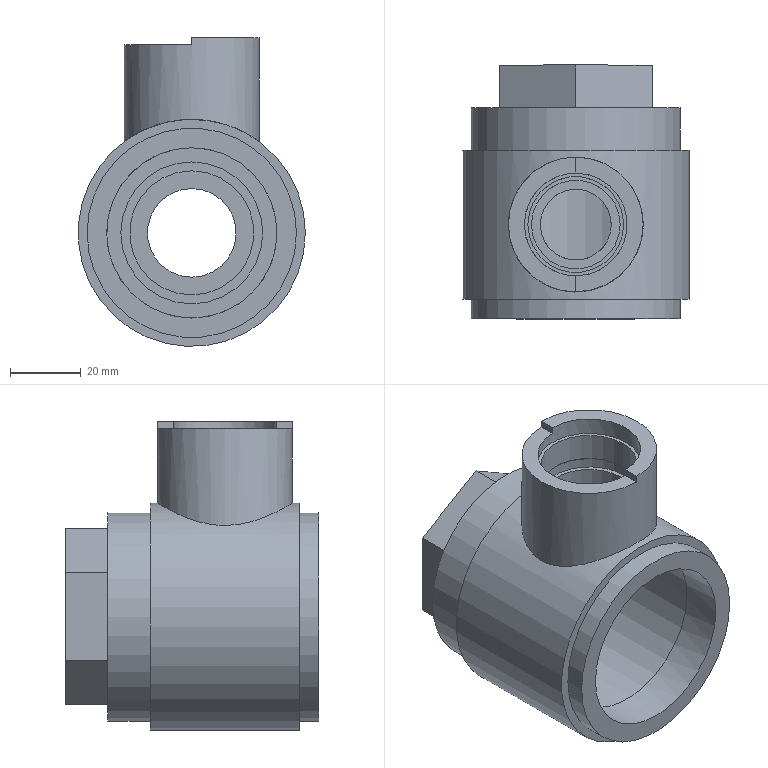Component | NX | VALVEBODY | 1 solid | 41 faces | volume 111936 mm3 | plane 25 | cylinder 16 | commonest cylinder face diameters 25 x2 59 x2 50 x1 34 x1 35 x1 40 x1 64 x1 38 x1